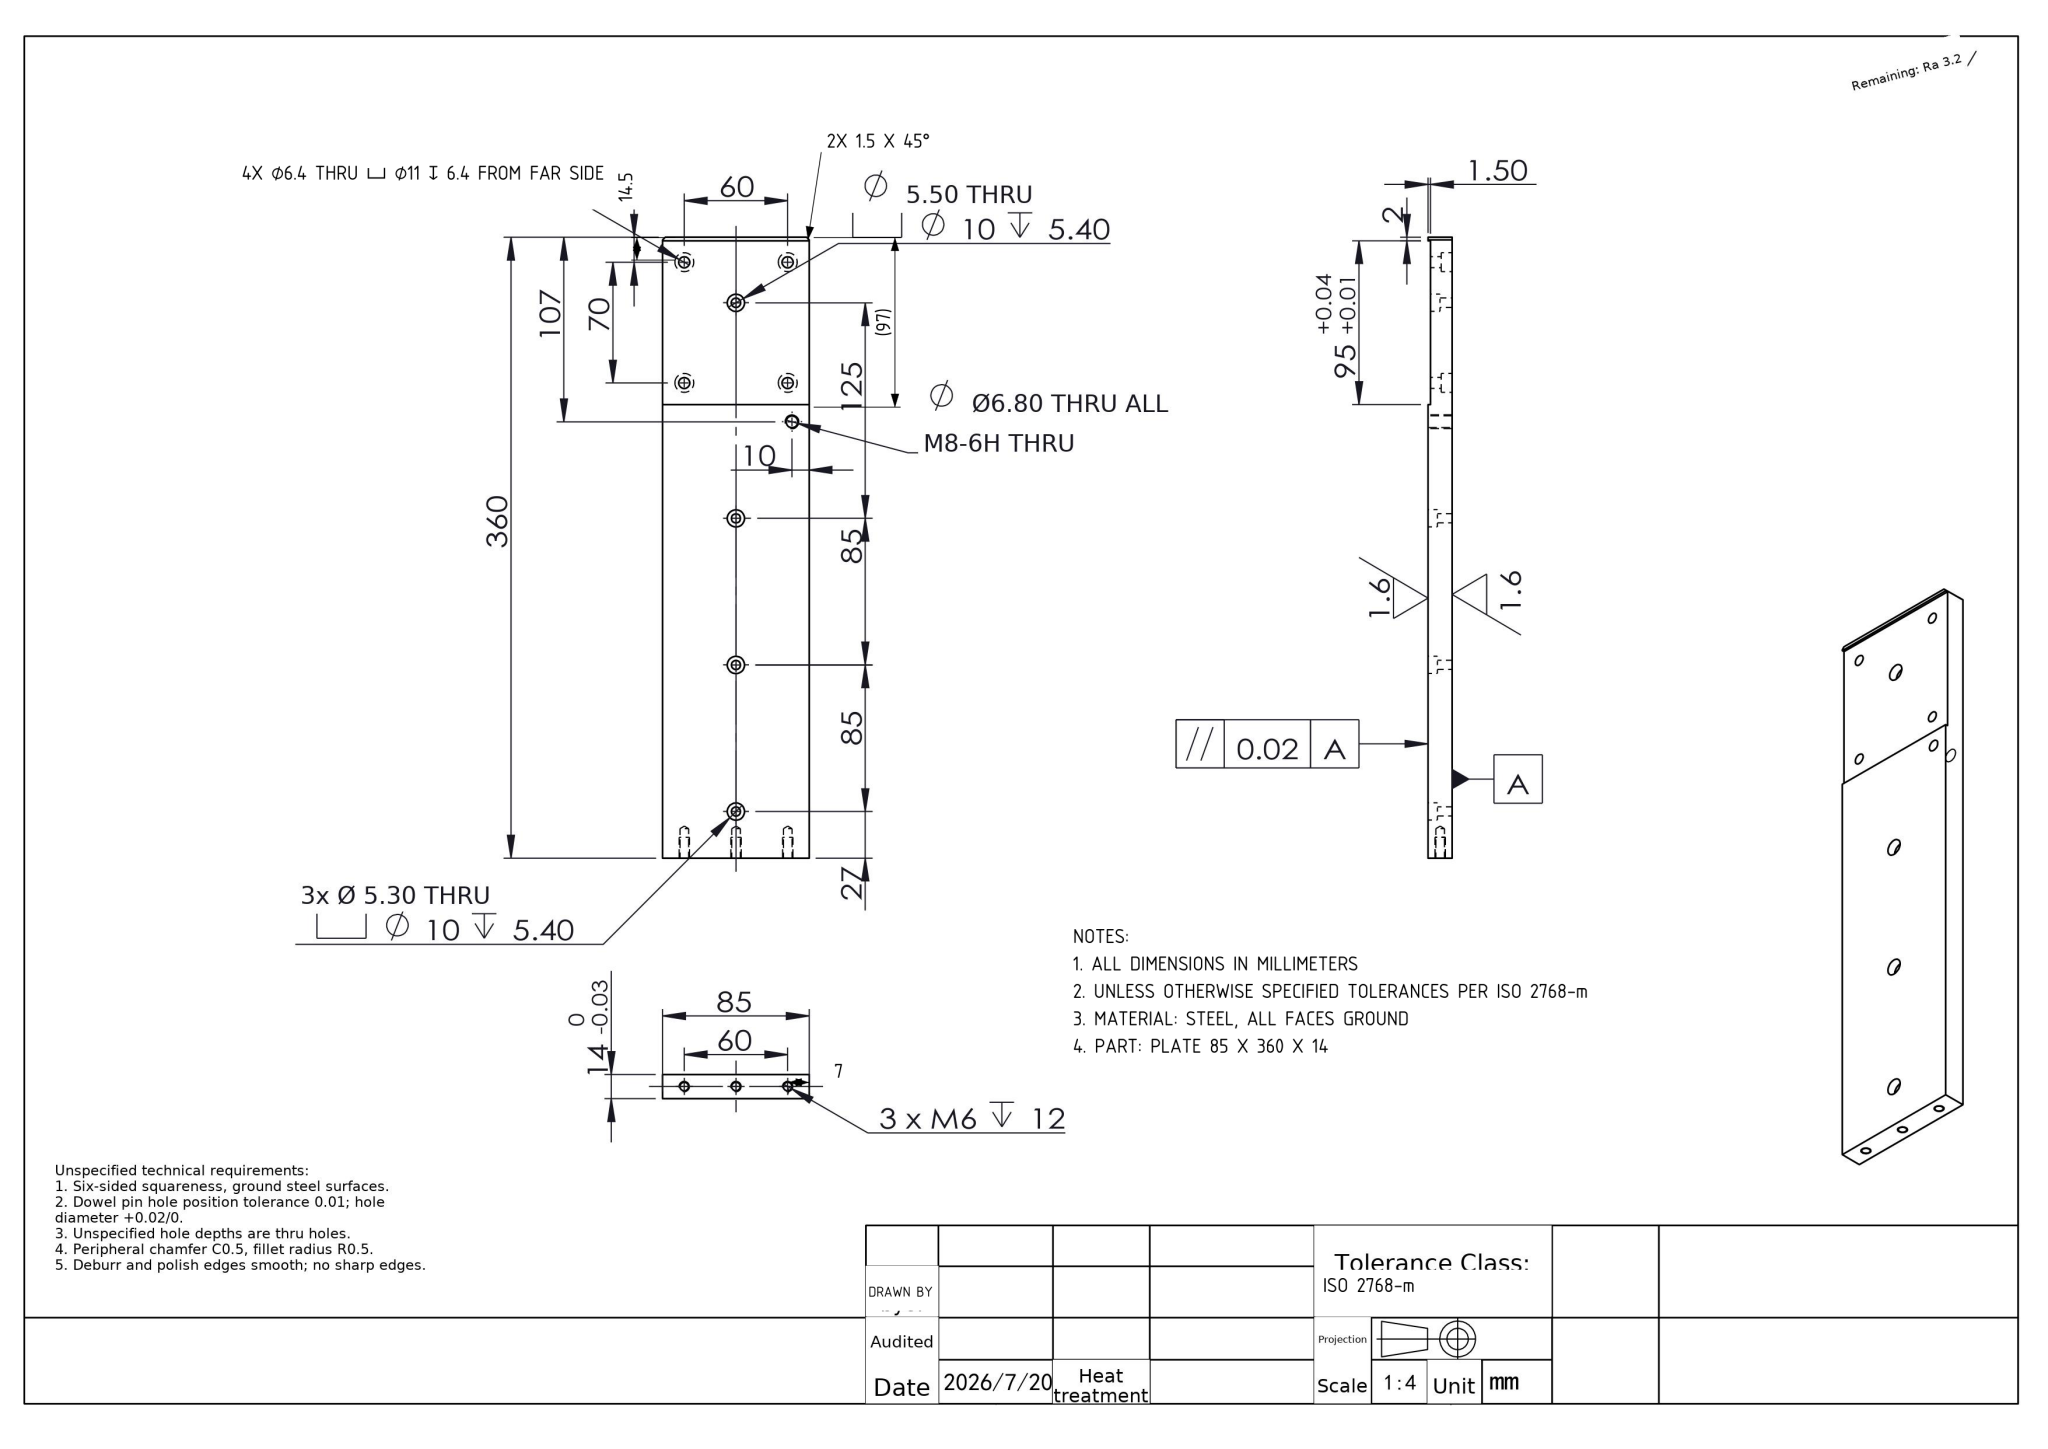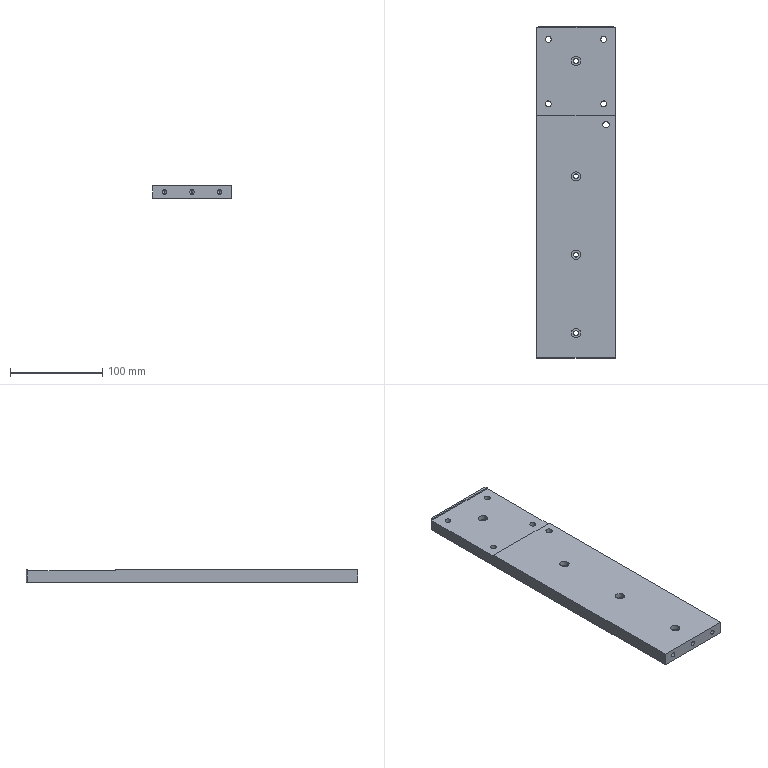Part | NX | mm | 1 solid | 66 faces | box 85 x 360 x 14 mm | volume 409065 mm3 | cylinder 40 | plane 20 | cone 6 | commonest cylinder face diameters 10 x8 11 x8 6.4 x8 5.3 x6 5 x6 6.8 x2 5.5 x2